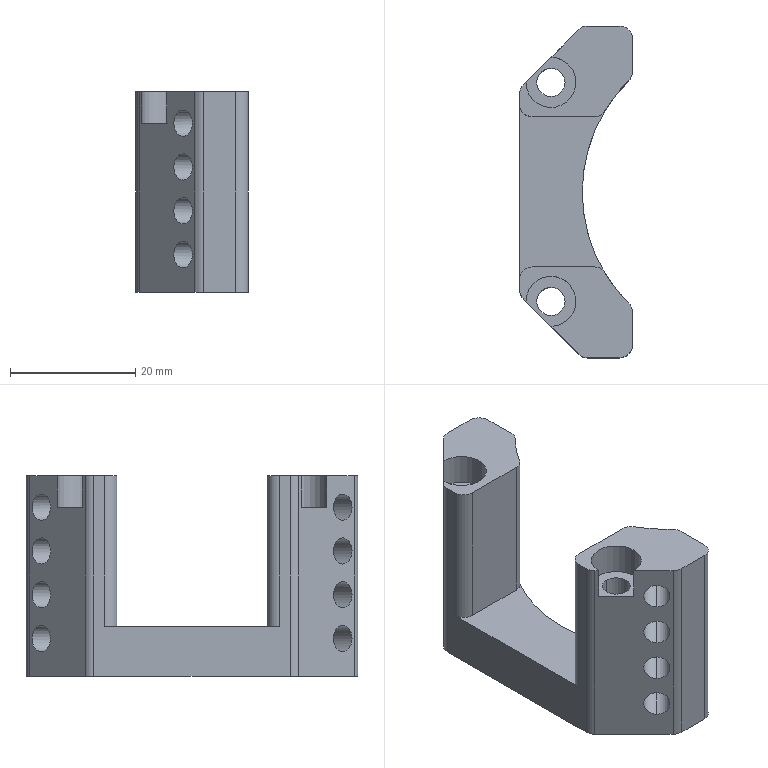CAM job | Mastercam | mm | 16 operations | part box 18 x 53 x 32
1. Facing | 24 - 100 平铣刀
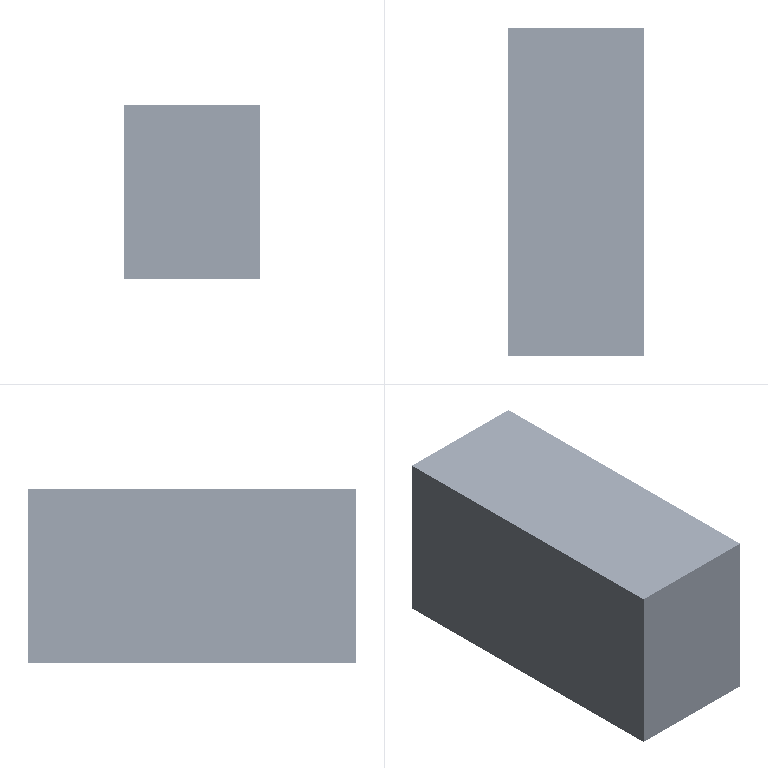2. 3D High Speed (Dynamic OptiRough) | 11 - 12 平铣刀
3. Contour (Ramp) | 4 - 4 平铣刀
4. Contour (2D) | 4 - 4 平铣刀
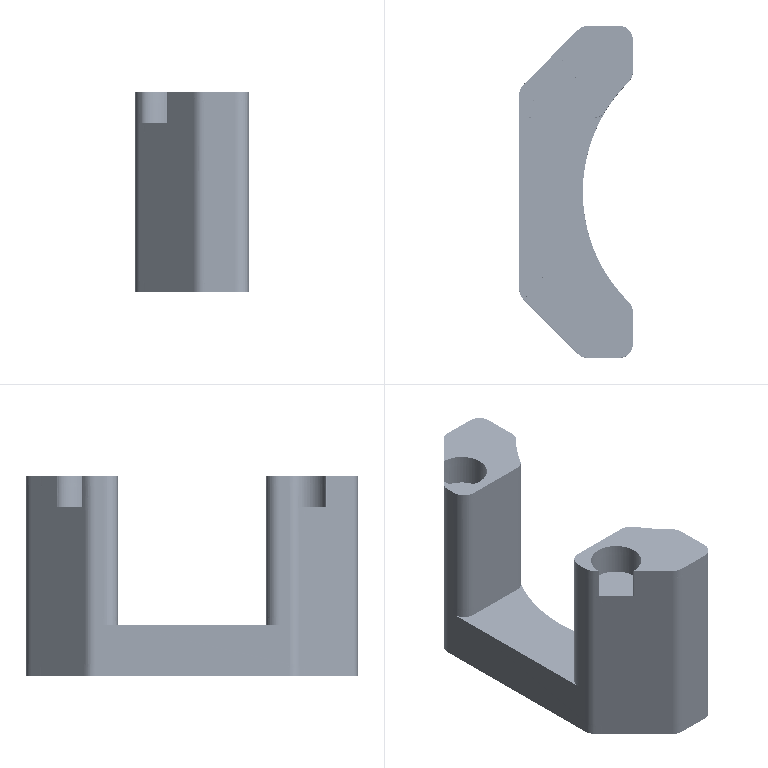5. 2D High Speed (2D Area Mill) | 12 - 12 平铣刀
6. Contour (2D) | 12 - 12 平铣刀
7. Contour (2D) | 12 - 12 平铣刀
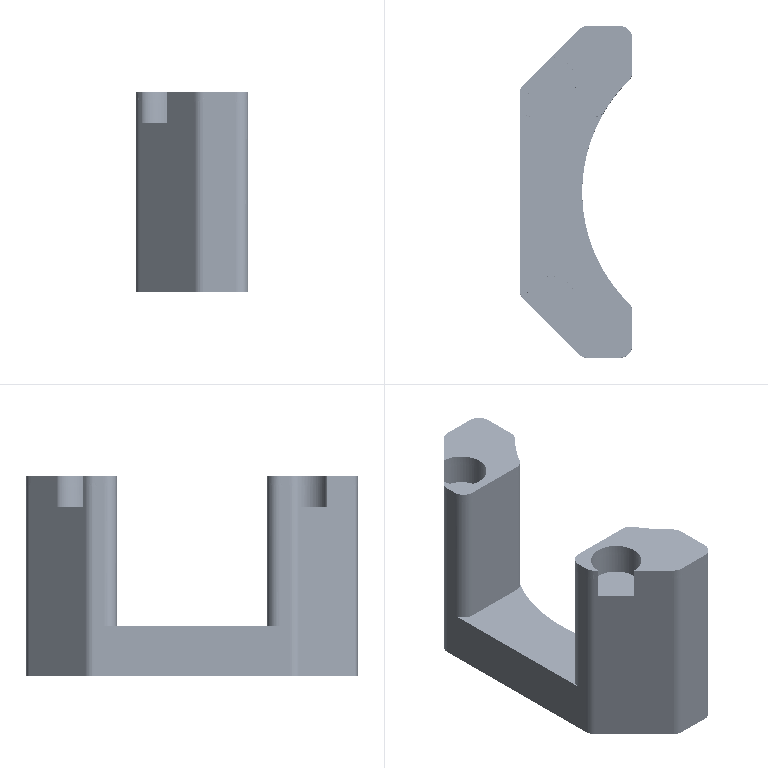8. Drill/Counterbore | 5 - 4 倒角刀
9. Contour (2D chamfer) | 5 - 4 倒角刀
10. 2D High Speed (2D Area Mill) | 4 - 4 平铣刀
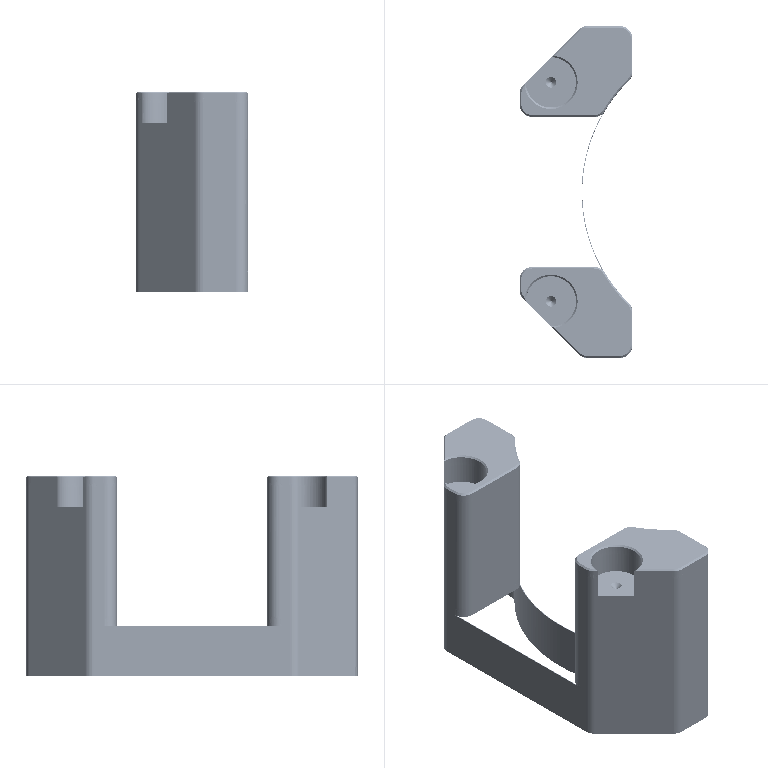11. Contour (2D) | 4 - 4 平铣刀
12. Contour (2D chamfer) | 5 - 4 倒角刀
13. Facing | 24 - 100 平铣刀
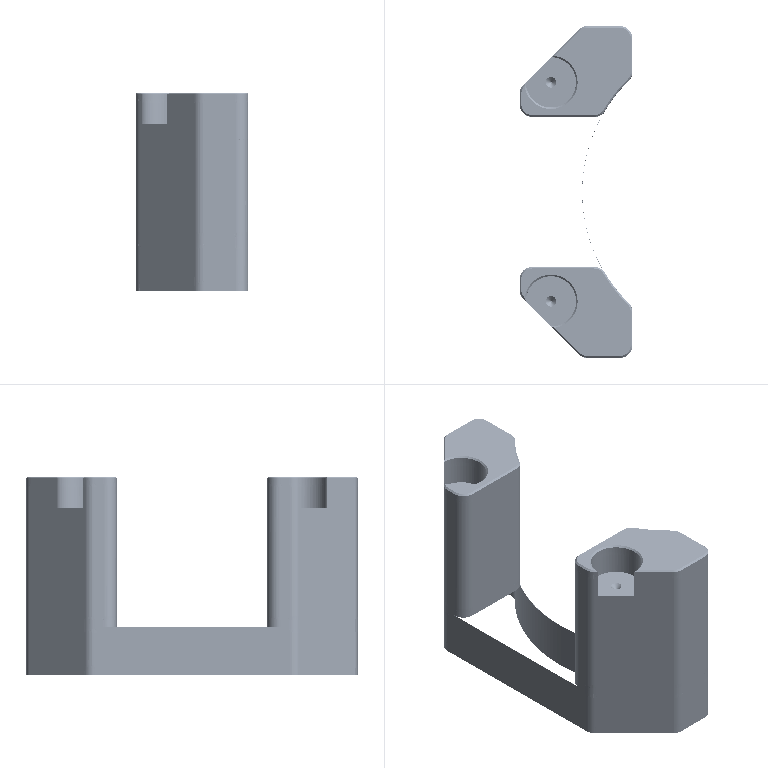14. Contour (2D chamfer) | 5 - 4 倒角刀
15. Drill/Counterbore | 5 - 4 倒角刀
16. Drill/Counterbore | 5 - 4 倒角刀